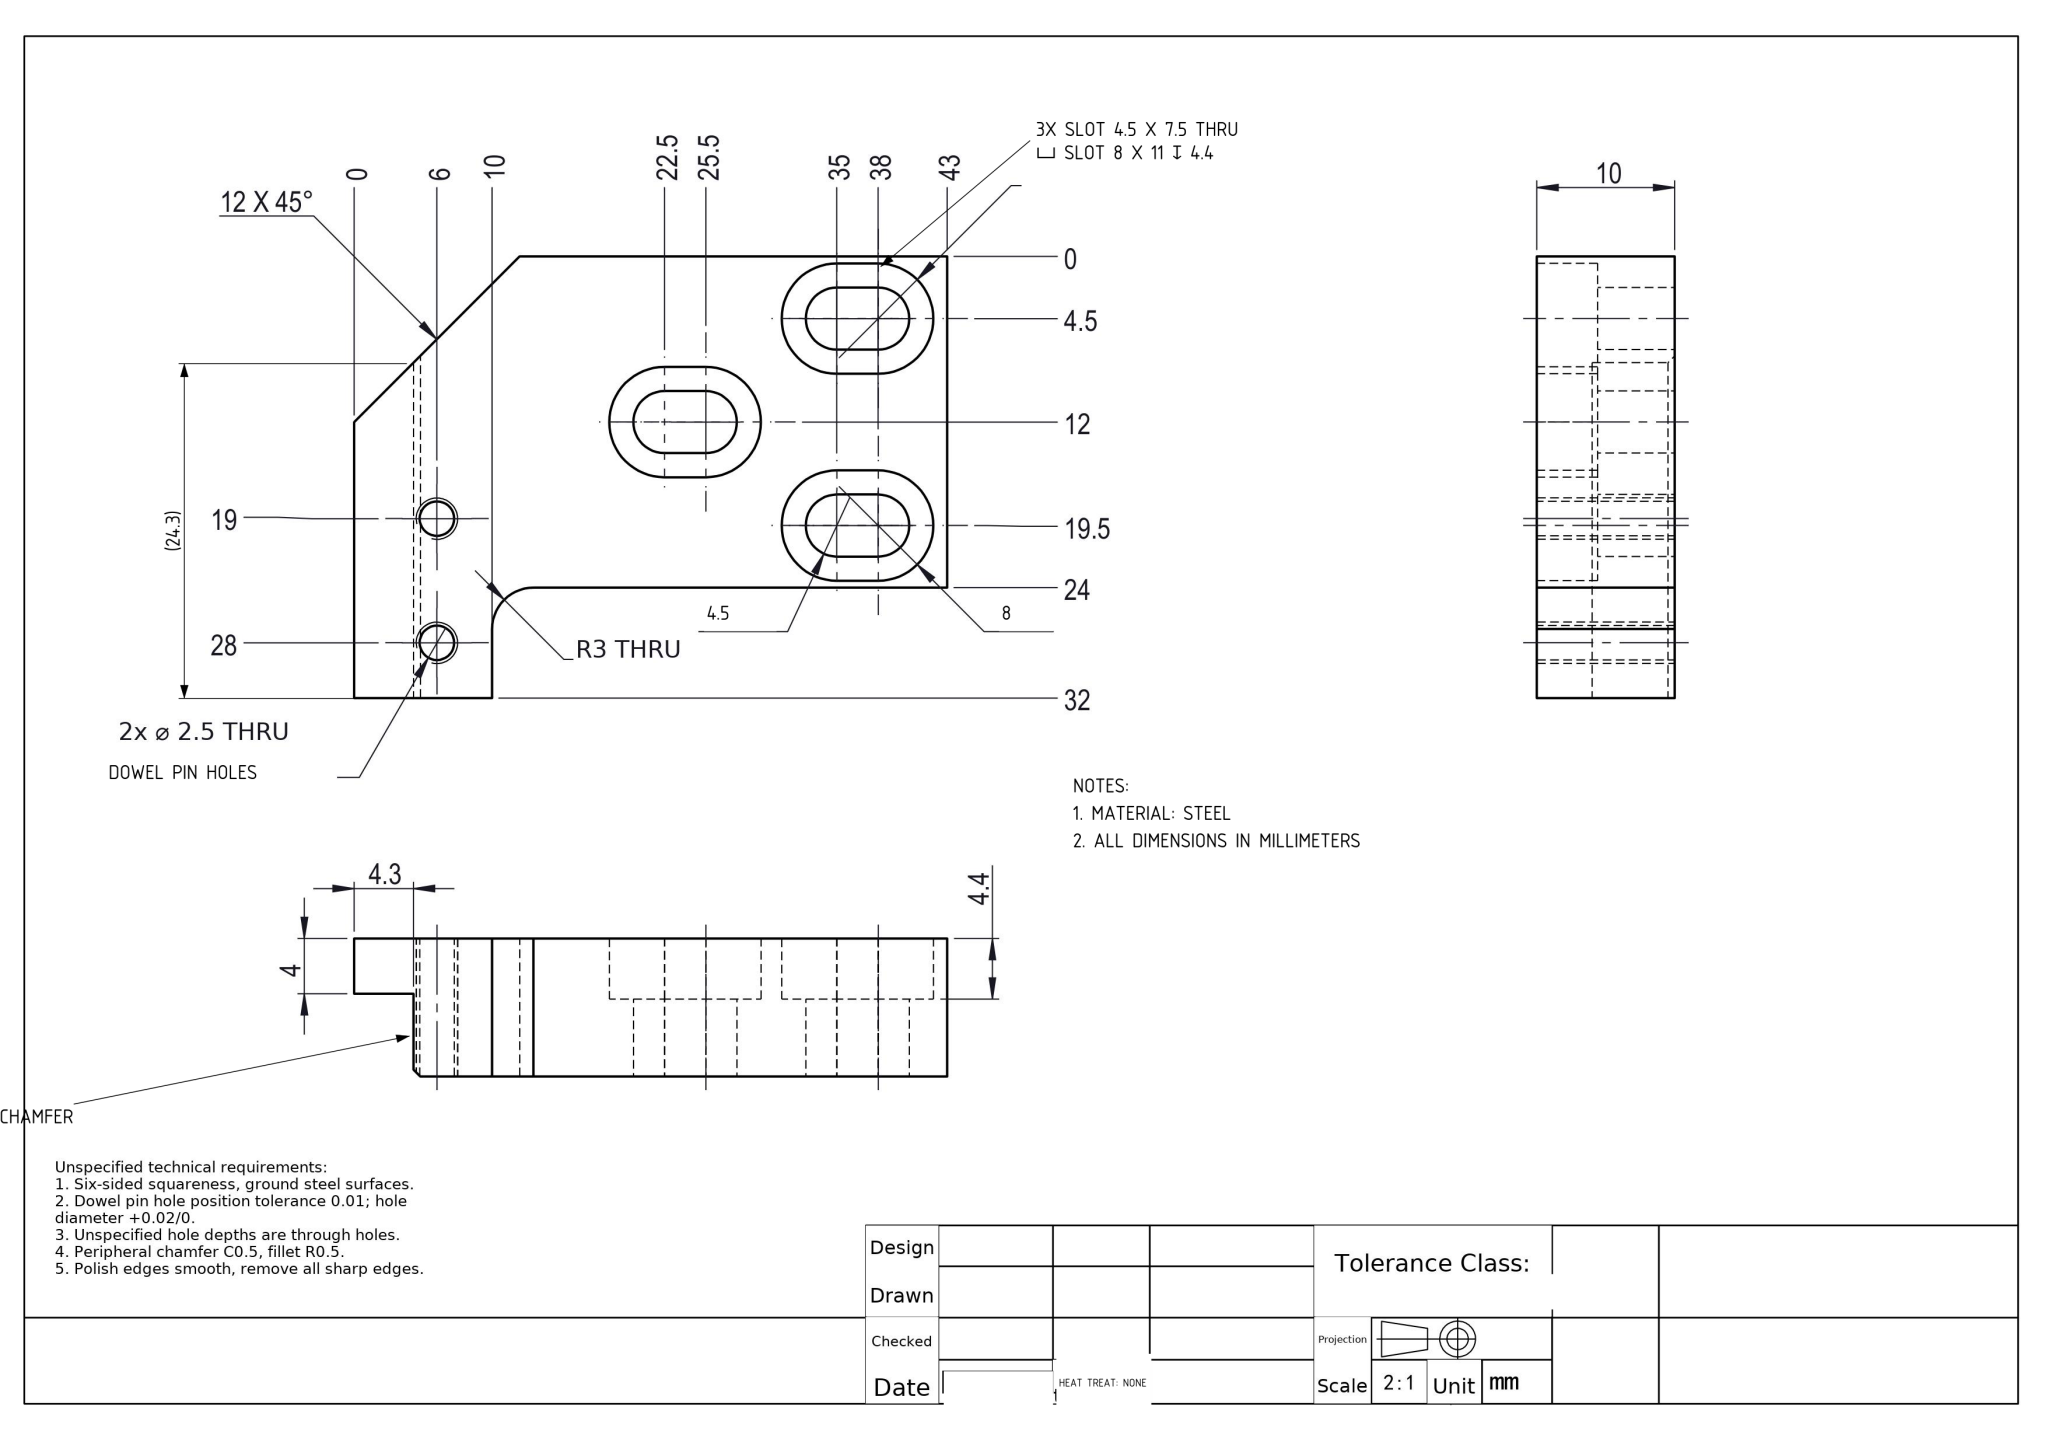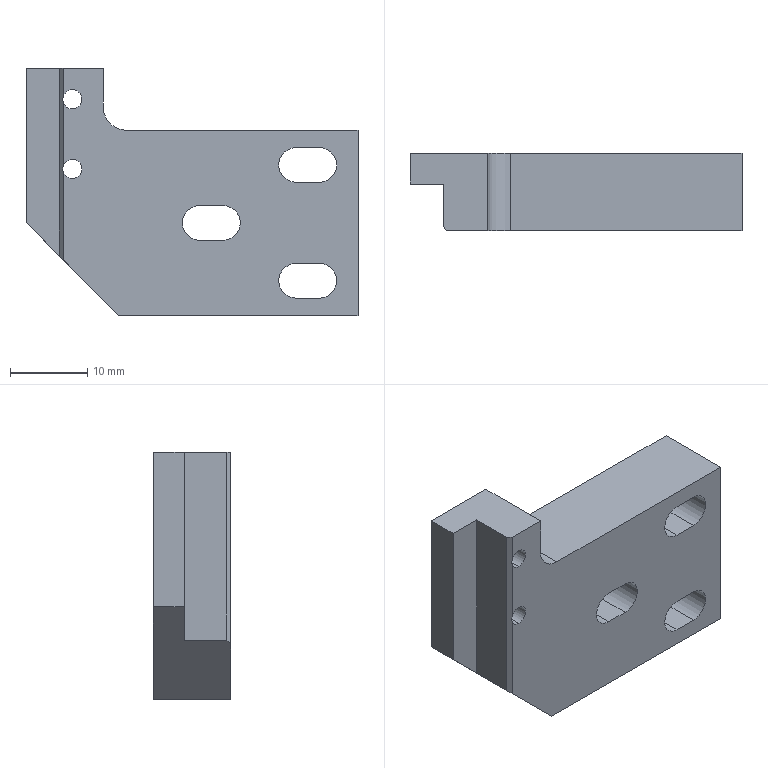Part | NX | mm | 1 solid | 44 faces | box 43 x 10 x 32 mm | volume 8272 mm3 | plane 27 | cylinder 17 | commonest cylinder face diameters 4.5 x6 8 x6 2.5 x4 6 x1